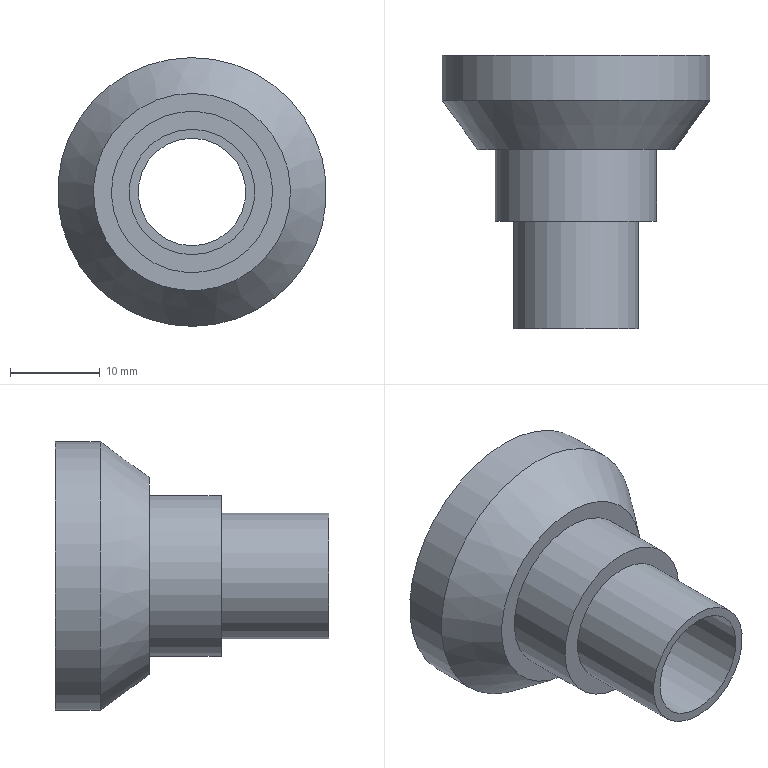Component | NX | 6 | 1 solid | 9 faces | box 30 x 30.5 x 30 mm | volume 6911 mm3 | plane 4 | cylinder 4 | cone 1 | commonest cylinder face diameters 12 x1 14 x1 18 x1 30 x1
STEP:
#1=CARTESIAN_POINT('',(0.,0.,0.));
#2=DIRECTION('',(0.,0.,1.));
#3=DIRECTION('',(1.,0.,0.));
#4=AXIS2_PLACEMENT_3D('',#1,#2,#3);
#5=CARTESIAN_POINT('',(-224.645,52.391,94.709));
#6=VERTEX_POINT('',#5);
#7=CARTESIAN_POINT('',(-221.817,52.391,100.));
#8=DIRECTION('',(0.,-1.,0.));
#9=DIRECTION('',(-0.4714,0.,-0.8819));
#10=AXIS2_PLACEMENT_3D('',#7,#8,#9);
#11=CIRCLE('',#10,6.);
#12=CARTESIAN_POINT('',(-208.588,52.391,92.928));
#13=DIRECTION('',(0.,1.,0.));
#14=DIRECTION('',(0.4714,0.,0.8819));
#15=AXIS2_PLACEMENT_3D('',#12,#13,#14);
#16=PLANE('',#15);
#17=CARTESIAN_POINT('',(-6.,-15.));
#18=CARTESIAN_POINT('',(-6.,-4.608));
#19=CARTESIAN_POINT('',(3.,-9.804));
#20=CARTESIAN_POINT('',(12.,-15.));
#21=CARTESIAN_POINT('',(3.,-20.196));
#22=CARTESIAN_POINT('',(-6.,-25.392));
#23=CARTESIAN_POINT('',(-6.,-15.));
#24=(BOUNDED_CURVE()B_SPLINE_CURVE(2,(#17,#18,#19,#20,#21,#22,#23),.UNSPECIFIED.,.T.,.F.)B_SPLINE_CURVE_WITH_KNOTS((1,2,2,2,2,1),(-2.094,0.,2.094,4.189,6.283,8.378),.UNSPECIFIED.)CURVE()GEOMETRIC_REPRESENTATION_ITEM()RATIONAL_B_SPLINE_CURVE((1.,0.5,1.,0.5,1.,0.5,1.))REPRESENTATION_ITEM(''));
#25=(GEOMETRIC_REPRESENTATION_CONTEXT(2)PARAMETRIC_REPRESENTATION_CONTEXT()REPRESENTATION_CONTEXT('',''));
#26=DEFINITIONAL_REPRESENTATION('',(#24),#25);
#27=PCURVE('',#16,#26);
#28=CARTESIAN_POINT('',(-221.817,52.391,100.));
#29=DIRECTION('',(0.,-1.,0.));
#30=DIRECTION('',(-0.4714,0.,-0.8819));
#31=AXIS2_PLACEMENT_3D('',#28,#29,#30);
#32=CYLINDRICAL_SURFACE('',#31,6.);
#33=CARTESIAN_POINT('',(0.,0.));
#34=DIRECTION('',(1.,0.));
#35=VECTOR('',#34,1.);
#36=LINE('',#33,#35);
#37=(GEOMETRIC_REPRESENTATION_CONTEXT(2)PARAMETRIC_REPRESENTATION_CONTEXT()REPRESENTATION_CONTEXT('',''));
#38=DEFINITIONAL_REPRESENTATION('',(#36),#37);
#39=PCURVE('',#32,#38);
#40=SURFACE_CURVE('',#11,(#27,#39),.PCURVE_S1.);
#41=EDGE_CURVE('',#6,#6,#40,.T.);
#42=ORIENTED_EDGE('',*,*,#41,.T.);
#43=EDGE_LOOP('',(#42));
#44=FACE_BOUND('',#43,.T.);
#45=CARTESIAN_POINT('',(-228.888,52.391,86.772));
#46=VERTEX_POINT('',#45);
#47=CARTESIAN_POINT('',(-221.817,52.391,100.));
#48=DIRECTION('',(0.,-1.,0.));
#49=DIRECTION('',(-0.4714,0.,-0.8819));
#50=AXIS2_PLACEMENT_3D('',#47,#48,#49);
#51=CIRCLE('',#50,15.);
#52=CARTESIAN_POINT('',(-15.,-15.));
#53=CARTESIAN_POINT('',(-15.,10.981));
#54=CARTESIAN_POINT('',(7.5,-2.01));
#55=CARTESIAN_POINT('',(30.,-15.));
#56=CARTESIAN_POINT('',(7.5,-27.99));
#57=CARTESIAN_POINT('',(-15.,-40.981));
#58=CARTESIAN_POINT('',(-15.,-15.));
#59=(BOUNDED_CURVE()B_SPLINE_CURVE(2,(#52,#53,#54,#55,#56,#57,#58),.UNSPECIFIED.,.T.,.F.)B_SPLINE_CURVE_WITH_KNOTS((1,2,2,2,2,1),(-2.094,0.,2.094,4.189,6.283,8.378),.UNSPECIFIED.)CURVE()GEOMETRIC_REPRESENTATION_ITEM()RATIONAL_B_SPLINE_CURVE((1.,0.5,1.,0.5,1.,0.5,1.))REPRESENTATION_ITEM(''));
#60=(GEOMETRIC_REPRESENTATION_CONTEXT(2)PARAMETRIC_REPRESENTATION_CONTEXT()REPRESENTATION_CONTEXT('',''));
#61=DEFINITIONAL_REPRESENTATION('',(#59),#60);
#62=PCURVE('',#16,#61);
#63=CARTESIAN_POINT('',(-221.817,52.391,100.));
#64=DIRECTION('',(0.,-1.,0.));
#65=DIRECTION('',(-0.4714,0.,-0.8819));
#66=AXIS2_PLACEMENT_3D('',#63,#64,#65);
#67=CYLINDRICAL_SURFACE('',#66,15.);
#68=CARTESIAN_POINT('',(0.,0.));
#69=DIRECTION('',(1.,0.));
#70=VECTOR('',#69,1.);
#71=LINE('',#68,#70);
#72=(GEOMETRIC_REPRESENTATION_CONTEXT(2)PARAMETRIC_REPRESENTATION_CONTEXT()REPRESENTATION_CONTEXT('',''));
#73=DEFINITIONAL_REPRESENTATION('',(#71),#72);
#74=PCURVE('',#67,#73);
#75=SURFACE_CURVE('',#51,(#62,#74),.PCURVE_S1.);
#76=EDGE_CURVE('',#46,#46,#75,.T.);
#77=ORIENTED_EDGE('',*,*,#76,.F.);
#78=EDGE_LOOP('',(#77));
#79=FACE_BOUND('',#78,.T.);
#80=ADVANCED_FACE('',(#44,#79),#16,.T.);
#81=CARTESIAN_POINT('',(-224.645,21.891,94.709));
#82=VERTEX_POINT('',#81);
#83=CARTESIAN_POINT('',(-221.817,21.891,100.));
#84=DIRECTION('',(0.,-1.,0.));
#85=DIRECTION('',(-0.4714,0.,-0.8819));
#86=AXIS2_PLACEMENT_3D('',#83,#84,#85);
#87=CIRCLE('',#86,6.);
#88=CARTESIAN_POINT('',(0.,30.5));
#89=DIRECTION('',(1.,0.));
#90=VECTOR('',#89,1.);
#91=LINE('',#88,#90);
#92=(GEOMETRIC_REPRESENTATION_CONTEXT(2)PARAMETRIC_REPRESENTATION_CONTEXT()REPRESENTATION_CONTEXT('',''));
#93=DEFINITIONAL_REPRESENTATION('',(#91),#92);
#94=PCURVE('',#32,#93);
#95=CARTESIAN_POINT('',(-216.525,21.891,97.171));
#96=DIRECTION('',(0.,-1.,0.));
#97=DIRECTION('',(-0.4714,0.,-0.8819));
#98=AXIS2_PLACEMENT_3D('',#95,#96,#97);
#99=PLANE('',#98);
#100=CARTESIAN_POINT('',(-0.,-6.));
#101=DIRECTION('',(1.,0.));
#102=AXIS2_PLACEMENT_2D('',#100,#101);
#103=CIRCLE('',#102,6.);
#104=(GEOMETRIC_REPRESENTATION_CONTEXT(2)PARAMETRIC_REPRESENTATION_CONTEXT()REPRESENTATION_CONTEXT('',''));
#105=DEFINITIONAL_REPRESENTATION('',(#103),#104);
#106=PCURVE('',#99,#105);
#107=SURFACE_CURVE('',#87,(#94,#106),.PCURVE_S1.);
#108=EDGE_CURVE('',#82,#82,#107,.T.);
#109=ORIENTED_EDGE('',*,*,#108,.F.);
#110=CARTESIAN_POINT('',(-224.645,52.391,94.709));
#111=CARTESIAN_POINT('',(-224.645,21.891,94.709));
#112=B_SPLINE_CURVE_WITH_KNOTS('',1,(#110,#111),.UNSPECIFIED.,.F.,.F.,(2,2),(0.,30.5),.PIECEWISE_BEZIER_KNOTS.);
#113=CARTESIAN_POINT('',(0.,0.));
#114=DIRECTION('',(0.,1.));
#115=VECTOR('',#114,1.);
#116=LINE('',#113,#115);
#117=(GEOMETRIC_REPRESENTATION_CONTEXT(2)PARAMETRIC_REPRESENTATION_CONTEXT()REPRESENTATION_CONTEXT('',''));
#118=DEFINITIONAL_REPRESENTATION('',(#116),#117);
#119=PCURVE('',#32,#118);
#120=CARTESIAN_POINT('',(6.283,0.));
#121=DIRECTION('',(0.,1.));
#122=VECTOR('',#121,1.);
#123=LINE('',#120,#122);
#124=(GEOMETRIC_REPRESENTATION_CONTEXT(2)PARAMETRIC_REPRESENTATION_CONTEXT()REPRESENTATION_CONTEXT('',''));
#125=DEFINITIONAL_REPRESENTATION('',(#123),#124);
#126=PCURVE('',#32,#125);
#127=SEAM_CURVE('',#112,(#119,#126),.PCURVE_S1.);
#128=EDGE_CURVE('',#6,#82,#127,.T.);
#129=ORIENTED_EDGE('',*,*,#128,.F.);
#130=ORIENTED_EDGE('',*,*,#41,.T.);
#131=ORIENTED_EDGE('',*,*,#128,.T.);
#132=EDGE_LOOP('',(#109,#129,#130,#131));
#133=FACE_BOUND('',#132,.F.);
#134=ADVANCED_FACE('',(#133),#32,.F.);
#135=CARTESIAN_POINT('',(-225.117,21.891,93.827));
#136=VERTEX_POINT('',#135);
#137=CARTESIAN_POINT('',(-221.817,21.891,100.));
#138=DIRECTION('',(0.,-1.,0.));
#139=DIRECTION('',(-0.4714,0.,-0.8819));
#140=AXIS2_PLACEMENT_3D('',#137,#138,#139);
#141=CIRCLE('',#140,7.);
#142=CARTESIAN_POINT('',(-0.,-6.));
#143=DIRECTION('',(1.,0.));
#144=AXIS2_PLACEMENT_2D('',#142,#143);
#145=CIRCLE('',#144,7.);
#146=(GEOMETRIC_REPRESENTATION_CONTEXT(2)PARAMETRIC_REPRESENTATION_CONTEXT()REPRESENTATION_CONTEXT('',''));
#147=DEFINITIONAL_REPRESENTATION('',(#145),#146);
#148=PCURVE('',#99,#147);
#149=CARTESIAN_POINT('',(-221.817,52.391,100.));
#150=DIRECTION('',(0.,-1.,0.));
#151=DIRECTION('',(-0.4714,0.,-0.8819));
#152=AXIS2_PLACEMENT_3D('',#149,#150,#151);
#153=CYLINDRICAL_SURFACE('',#152,7.);
#154=CARTESIAN_POINT('',(0.,30.5));
#155=DIRECTION('',(1.,0.));
#156=VECTOR('',#155,1.);
#157=LINE('',#154,#156);
#158=(GEOMETRIC_REPRESENTATION_CONTEXT(2)PARAMETRIC_REPRESENTATION_CONTEXT()REPRESENTATION_CONTEXT('',''));
#159=DEFINITIONAL_REPRESENTATION('',(#157),#158);
#160=PCURVE('',#153,#159);
#161=SURFACE_CURVE('',#141,(#148,#160),.PCURVE_S1.);
#162=EDGE_CURVE('',#136,#136,#161,.T.);
#163=ORIENTED_EDGE('',*,*,#162,.T.);
#164=EDGE_LOOP('',(#163));
#165=FACE_BOUND('',#164,.T.);
#166=ORIENTED_EDGE('',*,*,#108,.F.);
#167=EDGE_LOOP('',(#166));
#168=FACE_BOUND('',#167,.T.);
#169=ADVANCED_FACE('',(#165,#168),#99,.T.);
#170=CARTESIAN_POINT('',(-225.117,33.891,93.827));
#171=VERTEX_POINT('',#170);
#172=CARTESIAN_POINT('',(-221.817,33.891,100.));
#173=DIRECTION('',(0.,-1.,0.));
#174=DIRECTION('',(-0.4714,0.,-0.8819));
#175=AXIS2_PLACEMENT_3D('',#172,#173,#174);
#176=CIRCLE('',#175,7.);
#177=CARTESIAN_POINT('',(0.,18.5));
#178=DIRECTION('',(1.,0.));
#179=VECTOR('',#178,1.);
#180=LINE('',#177,#179);
#181=(GEOMETRIC_REPRESENTATION_CONTEXT(2)PARAMETRIC_REPRESENTATION_CONTEXT()REPRESENTATION_CONTEXT('',''));
#182=DEFINITIONAL_REPRESENTATION('',(#180),#181);
#183=PCURVE('',#153,#182);
#184=CARTESIAN_POINT('',(-215.643,33.891,96.7));
#185=DIRECTION('',(0.,-1.,0.));
#186=DIRECTION('',(-0.4714,0.,-0.8819));
#187=AXIS2_PLACEMENT_3D('',#184,#185,#186);
#188=PLANE('',#187);
#189=CARTESIAN_POINT('',(0.,-7.));
#190=DIRECTION('',(1.,0.));
#191=AXIS2_PLACEMENT_2D('',#189,#190);
#192=CIRCLE('',#191,7.);
#193=(GEOMETRIC_REPRESENTATION_CONTEXT(2)PARAMETRIC_REPRESENTATION_CONTEXT()REPRESENTATION_CONTEXT('',''));
#194=DEFINITIONAL_REPRESENTATION('',(#192),#193);
#195=PCURVE('',#188,#194);
#196=SURFACE_CURVE('',#176,(#183,#195),.PCURVE_S1.);
#197=EDGE_CURVE('',#171,#171,#196,.T.);
#198=ORIENTED_EDGE('',*,*,#197,.T.);
#199=CARTESIAN_POINT('',(-225.117,33.891,93.827));
#200=CARTESIAN_POINT('',(-225.117,21.891,93.827));
#201=B_SPLINE_CURVE_WITH_KNOTS('',1,(#199,#200),.UNSPECIFIED.,.F.,.F.,(2,2),(18.5,30.5),.PIECEWISE_BEZIER_KNOTS.);
#202=CARTESIAN_POINT('',(6.283,0.));
#203=DIRECTION('',(0.,1.));
#204=VECTOR('',#203,1.);
#205=LINE('',#202,#204);
#206=(GEOMETRIC_REPRESENTATION_CONTEXT(2)PARAMETRIC_REPRESENTATION_CONTEXT()REPRESENTATION_CONTEXT('',''));
#207=DEFINITIONAL_REPRESENTATION('',(#205),#206);
#208=PCURVE('',#153,#207);
#209=CARTESIAN_POINT('',(0.,0.));
#210=DIRECTION('',(0.,1.));
#211=VECTOR('',#210,1.);
#212=LINE('',#209,#211);
#213=(GEOMETRIC_REPRESENTATION_CONTEXT(2)PARAMETRIC_REPRESENTATION_CONTEXT()REPRESENTATION_CONTEXT('',''));
#214=DEFINITIONAL_REPRESENTATION('',(#212),#213);
#215=PCURVE('',#153,#214);
#216=SEAM_CURVE('',#201,(#208,#215),.PCURVE_S1.);
#217=EDGE_CURVE('',#171,#136,#216,.T.);
#218=ORIENTED_EDGE('',*,*,#217,.T.);
#219=ORIENTED_EDGE('',*,*,#162,.F.);
#220=ORIENTED_EDGE('',*,*,#217,.F.);
#221=EDGE_LOOP('',(#198,#218,#219,#220));
#222=FACE_BOUND('',#221,.T.);
#223=ADVANCED_FACE('',(#222),#153,.T.);
#224=CARTESIAN_POINT('',(-226.06,33.891,92.063));
#225=VERTEX_POINT('',#224);
#226=CARTESIAN_POINT('',(-221.817,33.891,100.));
#227=DIRECTION('',(0.,-1.,0.));
#228=DIRECTION('',(-0.4714,0.,-0.8819));
#229=AXIS2_PLACEMENT_3D('',#226,#227,#228);
#230=CIRCLE('',#229,9.);
#231=CARTESIAN_POINT('',(0.,-7.));
#232=DIRECTION('',(1.,0.));
#233=AXIS2_PLACEMENT_2D('',#231,#232);
#234=CIRCLE('',#233,9.);
#235=(GEOMETRIC_REPRESENTATION_CONTEXT(2)PARAMETRIC_REPRESENTATION_CONTEXT()REPRESENTATION_CONTEXT('',''));
#236=DEFINITIONAL_REPRESENTATION('',(#234),#235);
#237=PCURVE('',#188,#236);
#238=CARTESIAN_POINT('',(-221.817,52.391,100.));
#239=DIRECTION('',(0.,-1.,0.));
#240=DIRECTION('',(-0.4714,0.,-0.8819));
#241=AXIS2_PLACEMENT_3D('',#238,#239,#240);
#242=CYLINDRICAL_SURFACE('',#241,9.);
#243=CARTESIAN_POINT('',(0.,18.5));
#244=DIRECTION('',(1.,0.));
#245=VECTOR('',#244,1.);
#246=LINE('',#243,#245);
#247=(GEOMETRIC_REPRESENTATION_CONTEXT(2)PARAMETRIC_REPRESENTATION_CONTEXT()REPRESENTATION_CONTEXT('',''));
#248=DEFINITIONAL_REPRESENTATION('',(#246),#247);
#249=PCURVE('',#242,#248);
#250=SURFACE_CURVE('',#230,(#237,#249),.PCURVE_S1.);
#251=EDGE_CURVE('',#225,#225,#250,.T.);
#252=ORIENTED_EDGE('',*,*,#251,.T.);
#253=EDGE_LOOP('',(#252));
#254=FACE_BOUND('',#253,.T.);
#255=ORIENTED_EDGE('',*,*,#197,.F.);
#256=EDGE_LOOP('',(#255));
#257=FACE_BOUND('',#256,.T.);
#258=ADVANCED_FACE('',(#254,#257),#188,.T.);
#259=CARTESIAN_POINT('',(-226.06,41.891,92.063));
#260=VERTEX_POINT('',#259);
#261=CARTESIAN_POINT('',(-221.817,41.891,100.));
#262=DIRECTION('',(0.,-1.,0.));
#263=DIRECTION('',(-0.4714,0.,-0.8819));
#264=AXIS2_PLACEMENT_3D('',#261,#262,#263);
#265=CIRCLE('',#264,9.);
#266=CARTESIAN_POINT('',(0.,10.5));
#267=DIRECTION('',(1.,0.));
#268=VECTOR('',#267,1.);
#269=LINE('',#266,#268);
#270=(GEOMETRIC_REPRESENTATION_CONTEXT(2)PARAMETRIC_REPRESENTATION_CONTEXT()REPRESENTATION_CONTEXT('',''));
#271=DEFINITIONAL_REPRESENTATION('',(#269),#270);
#272=PCURVE('',#242,#271);
#273=CARTESIAN_POINT('',(-213.88,41.891,95.757));
#274=DIRECTION('',(0.,-1.,0.));
#275=DIRECTION('',(-0.4714,0.,-0.8819));
#276=AXIS2_PLACEMENT_3D('',#273,#274,#275);
#277=PLANE('',#276);
#278=CARTESIAN_POINT('',(-0.,-9.));
#279=DIRECTION('',(1.,0.));
#280=AXIS2_PLACEMENT_2D('',#278,#279);
#281=CIRCLE('',#280,9.);
#282=(GEOMETRIC_REPRESENTATION_CONTEXT(2)PARAMETRIC_REPRESENTATION_CONTEXT()REPRESENTATION_CONTEXT('',''));
#283=DEFINITIONAL_REPRESENTATION('',(#281),#282);
#284=PCURVE('',#277,#283);
#285=SURFACE_CURVE('',#265,(#272,#284),.PCURVE_S1.);
#286=EDGE_CURVE('',#260,#260,#285,.T.);
#287=ORIENTED_EDGE('',*,*,#286,.T.);
#288=CARTESIAN_POINT('',(-226.06,41.891,92.063));
#289=CARTESIAN_POINT('',(-226.06,33.891,92.063));
#290=B_SPLINE_CURVE_WITH_KNOTS('',1,(#288,#289),.UNSPECIFIED.,.F.,.F.,(2,2),(10.5,18.5),.PIECEWISE_BEZIER_KNOTS.);
#291=CARTESIAN_POINT('',(6.283,0.));
#292=DIRECTION('',(0.,1.));
#293=VECTOR('',#292,1.);
#294=LINE('',#291,#293);
#295=(GEOMETRIC_REPRESENTATION_CONTEXT(2)PARAMETRIC_REPRESENTATION_CONTEXT()REPRESENTATION_CONTEXT('',''));
#296=DEFINITIONAL_REPRESENTATION('',(#294),#295);
#297=PCURVE('',#242,#296);
#298=CARTESIAN_POINT('',(0.,0.));
#299=DIRECTION('',(0.,1.));
#300=VECTOR('',#299,1.);
#301=LINE('',#298,#300);
#302=(GEOMETRIC_REPRESENTATION_CONTEXT(2)PARAMETRIC_REPRESENTATION_CONTEXT()REPRESENTATION_CONTEXT('',''));
#303=DEFINITIONAL_REPRESENTATION('',(#301),#302);
#304=PCURVE('',#242,#303);
#305=SEAM_CURVE('',#290,(#297,#304),.PCURVE_S1.);
#306=EDGE_CURVE('',#260,#225,#305,.T.);
#307=ORIENTED_EDGE('',*,*,#306,.T.);
#308=ORIENTED_EDGE('',*,*,#251,.F.);
#309=ORIENTED_EDGE('',*,*,#306,.F.);
#310=EDGE_LOOP('',(#287,#307,#308,#309));
#311=FACE_BOUND('',#310,.T.);
#312=ADVANCED_FACE('',(#311),#242,.T.);
#313=CARTESIAN_POINT('',(-227.003,41.891,90.299));
#314=VERTEX_POINT('',#313);
#315=CARTESIAN_POINT('',(-221.817,41.891,100.));
#316=DIRECTION('',(0.,-1.,0.));
#317=DIRECTION('',(-0.4714,0.,-0.8819));
#318=AXIS2_PLACEMENT_3D('',#315,#316,#317);
#319=CIRCLE('',#318,11.);
#320=CARTESIAN_POINT('',(-0.,-9.));
#321=DIRECTION('',(1.,0.));
#322=AXIS2_PLACEMENT_2D('',#320,#321);
#323=CIRCLE('',#322,11.);
#324=(GEOMETRIC_REPRESENTATION_CONTEXT(2)PARAMETRIC_REPRESENTATION_CONTEXT()REPRESENTATION_CONTEXT('',''));
#325=DEFINITIONAL_REPRESENTATION('',(#323),#324);
#326=PCURVE('',#277,#325);
#327=CARTESIAN_POINT('',(-221.817,41.891,100.));
#328=DIRECTION('',(0.,1.,0.));
#329=DIRECTION('',(0.4714,0.,0.8819));
#330=AXIS2_PLACEMENT_3D('',#327,#328,#329);
#331=CONICAL_SURFACE('',#330,11.,0.6288);
#332=CARTESIAN_POINT('',(9.425,0.));
#333=DIRECTION('',(-1.,0.));
#334=VECTOR('',#333,1.);
#335=LINE('',#332,#334);
#336=(GEOMETRIC_REPRESENTATION_CONTEXT(2)PARAMETRIC_REPRESENTATION_CONTEXT()REPRESENTATION_CONTEXT('',''));
#337=DEFINITIONAL_REPRESENTATION('',(#335),#336);
#338=PCURVE('',#331,#337);
#339=SURFACE_CURVE('',#319,(#326,#338),.PCURVE_S1.);
#340=EDGE_CURVE('',#314,#314,#339,.T.);
#341=ORIENTED_EDGE('',*,*,#340,.T.);
#342=EDGE_LOOP('',(#341));
#343=FACE_BOUND('',#342,.T.);
#344=ORIENTED_EDGE('',*,*,#286,.F.);
#345=EDGE_LOOP('',(#344));
#346=FACE_BOUND('',#345,.T.);
#347=ADVANCED_FACE('',(#343,#346),#277,.T.);
#348=CARTESIAN_POINT('',(-228.888,47.391,86.772));
#349=VERTEX_POINT('',#348);
#350=CARTESIAN_POINT('',(-221.817,47.391,100.));
#351=DIRECTION('',(0.,-1.,0.));
#352=DIRECTION('',(-0.4714,0.,-0.8819));
#353=AXIS2_PLACEMENT_3D('',#350,#351,#352);
#354=CIRCLE('',#353,15.);
#355=CARTESIAN_POINT('',(9.425,5.5));
#356=DIRECTION('',(-1.,-0.));
#357=VECTOR('',#356,1.);
#358=LINE('',#355,#357);
#359=(GEOMETRIC_REPRESENTATION_CONTEXT(2)PARAMETRIC_REPRESENTATION_CONTEXT()REPRESENTATION_CONTEXT('',''));
#360=DEFINITIONAL_REPRESENTATION('',(#358),#359);
#361=PCURVE('',#331,#360);
#362=CARTESIAN_POINT('',(0.,5.));
#363=DIRECTION('',(1.,0.));
#364=VECTOR('',#363,1.);
#365=LINE('',#362,#364);
#366=(GEOMETRIC_REPRESENTATION_CONTEXT(2)PARAMETRIC_REPRESENTATION_CONTEXT()REPRESENTATION_CONTEXT('',''));
#367=DEFINITIONAL_REPRESENTATION('',(#365),#366);
#368=PCURVE('',#67,#367);
#369=SURFACE_CURVE('',#354,(#361,#368),.PCURVE_S1.);
#370=EDGE_CURVE('',#349,#349,#369,.T.);
#371=ORIENTED_EDGE('',*,*,#370,.T.);
#372=CARTESIAN_POINT('',(-227.003,41.891,90.299));
#373=CARTESIAN_POINT('',(-228.888,47.391,86.772));
#374=B_SPLINE_CURVE_WITH_KNOTS('',1,(#372,#373),.UNSPECIFIED.,.F.,.F.,(2,2),(0.,6.801),.PIECEWISE_BEZIER_KNOTS.);
#375=CARTESIAN_POINT('',(3.142,0.));
#376=DIRECTION('',(0.,1.));
#377=VECTOR('',#376,1.);
#378=LINE('',#375,#377);
#379=(GEOMETRIC_REPRESENTATION_CONTEXT(2)PARAMETRIC_REPRESENTATION_CONTEXT()REPRESENTATION_CONTEXT('',''));
#380=DEFINITIONAL_REPRESENTATION('',(#378),#379);
#381=PCURVE('',#331,#380);
#382=CARTESIAN_POINT('',(9.425,0.));
#383=DIRECTION('',(0.,1.));
#384=VECTOR('',#383,1.);
#385=LINE('',#382,#384);
#386=(GEOMETRIC_REPRESENTATION_CONTEXT(2)PARAMETRIC_REPRESENTATION_CONTEXT()REPRESENTATION_CONTEXT('',''));
#387=DEFINITIONAL_REPRESENTATION('',(#385),#386);
#388=PCURVE('',#331,#387);
#389=SEAM_CURVE('',#374,(#381,#388),.PCURVE_S1.);
#390=EDGE_CURVE('',#314,#349,#389,.T.);
#391=ORIENTED_EDGE('',*,*,#390,.F.);
#392=ORIENTED_EDGE('',*,*,#340,.F.);
#393=ORIENTED_EDGE('',*,*,#390,.T.);
#394=EDGE_LOOP('',(#371,#391,#392,#393));
#395=FACE_BOUND('',#394,.T.);
#396=ADVANCED_FACE('',(#395),#331,.T.);
#397=ORIENTED_EDGE('',*,*,#76,.T.);
#398=CARTESIAN_POINT('',(-228.888,52.391,86.772));
#399=CARTESIAN_POINT('',(-228.888,47.391,86.772));
#400=B_SPLINE_CURVE_WITH_KNOTS('',1,(#398,#399),.UNSPECIFIED.,.F.,.F.,(2,2),(0.,5.),.PIECEWISE_BEZIER_KNOTS.);
#401=CARTESIAN_POINT('',(6.283,0.));
#402=DIRECTION('',(0.,1.));
#403=VECTOR('',#402,1.);
#404=LINE('',#401,#403);
#405=(GEOMETRIC_REPRESENTATION_CONTEXT(2)PARAMETRIC_REPRESENTATION_CONTEXT()REPRESENTATION_CONTEXT('',''));
#406=DEFINITIONAL_REPRESENTATION('',(#404),#405);
#407=PCURVE('',#67,#406);
#408=CARTESIAN_POINT('',(0.,0.));
#409=DIRECTION('',(0.,1.));
#410=VECTOR('',#409,1.);
#411=LINE('',#408,#410);
#412=(GEOMETRIC_REPRESENTATION_CONTEXT(2)PARAMETRIC_REPRESENTATION_CONTEXT()REPRESENTATION_CONTEXT('',''));
#413=DEFINITIONAL_REPRESENTATION('',(#411),#412);
#414=PCURVE('',#67,#413);
#415=SEAM_CURVE('',#400,(#407,#414),.PCURVE_S1.);
#416=EDGE_CURVE('',#46,#349,#415,.T.);
#417=ORIENTED_EDGE('',*,*,#416,.T.);
#418=ORIENTED_EDGE('',*,*,#370,.F.);
#419=ORIENTED_EDGE('',*,*,#416,.F.);
#420=EDGE_LOOP('',(#397,#417,#418,#419));
#421=FACE_BOUND('',#420,.T.);
#422=ADVANCED_FACE('',(#421),#67,.T.);
#423=CLOSED_SHELL('',(#80,#134,#169,#223,#258,#312,#347,#396,#422));
#424=MANIFOLD_SOLID_BREP('',#423);
#425=(LENGTH_UNIT()NAMED_UNIT(*)SI_UNIT(.MILLI.,.METRE.));
#426=UNCERTAINTY_MEASURE_WITH_UNIT(LENGTH_MEASURE(0.00001),#425,'','');
#427=(NAMED_UNIT(*)PLANE_ANGLE_UNIT()SI_UNIT($,.RADIAN.));
#428=(NAMED_UNIT(*)SI_UNIT($,.STERADIAN.)SOLID_ANGLE_UNIT());
#429=(GEOMETRIC_REPRESENTATION_CONTEXT(3)GLOBAL_UNCERTAINTY_ASSIGNED_CONTEXT((#426))GLOBAL_UNIT_ASSIGNED_CONTEXT((#425,#427,#428))REPRESENTATION_CONTEXT('',''));
#430=ADVANCED_BREP_SHAPE_REPRESENTATION('',(#4,#424),#429);